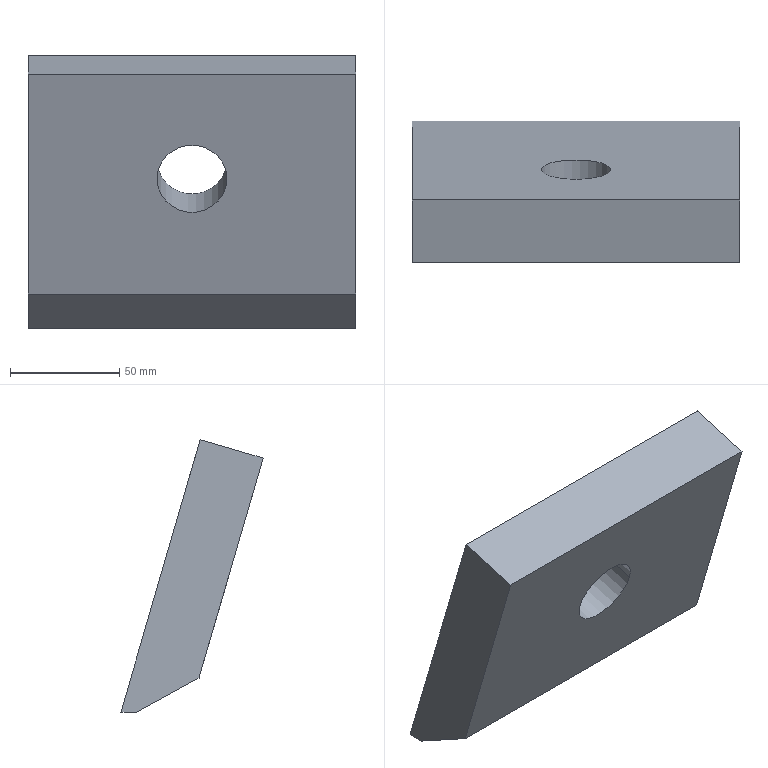Component | SolidWorks | Oslona ploca izbacivaca-4 | 1 solid | 9 faces | box 150 x 65.17 x 124.91 mm | volume 513260 mm3 | plane 6 | cylinder 3 | commonest cylinder face diameters 32 x2 521 x1
build123d program:
from build123d import *

# Parameters (mm, degrees)
SKETCH1_W           = 150
SKETCH1_H           = 130
SKETCH1_R           = 16
BOSS_EXTRUDE1_DEPTH = 30
CHAMFER1_SIZE       = 25
PIPECOPE_DEPTH      = 201.749
PIPECOPE_DEPTH_BACK = 201.749
PIPECOPESKETCH_R    = 260.5


with BuildPart() as part:
    # Sketch1 → Boss-Extrude1 (new body)
    with BuildSketch(Plane.XY):
        with Locations((75, 65)):
            Rectangle(SKETCH1_W, SKETCH1_H)
        with Locations((75, 80)):
            Circle(SKETCH1_R, mode=Mode.SUBTRACT)
    extrude(amount=BOSS_EXTRUDE1_DEPTH)

    # Chamfer1
    chamfer1_edges = [part.edges().sort_by_distance(p)[0] for p in [
        (75, 0, 0),
    ]]
    chamfer(chamfer1_edges, length=CHAMFER1_SIZE)

    # PipeCopeSketch → PipeCope (cut, two sides: drawn at the far end of the back side and taken through both)
    with BuildSketch(Plane(origin=(0, 0, 0), x_dir=(0, 0, -1), z_dir=(1, 0, 0)).offset(-PIPECOPE_DEPTH_BACK)):
        with Locations((42.874, -250.099)):
            Circle(PIPECOPESKETCH_R)
    extrude(amount=PIPECOPE_DEPTH + PIPECOPE_DEPTH_BACK, mode=Mode.SUBTRACT)


solid = part.part

# Placed as in the assembly
solid = solid.moved(Location((0.0002347, -28.803, 252.108), (-73.755, 0, 180)))
STEP:
#1=COLOUR_RGB('',0.7922,0.8196,0.9333);
#2=FILL_AREA_STYLE_COLOUR('',#1);
#3=FILL_AREA_STYLE('',(#2));
#4=SURFACE_STYLE_FILL_AREA(#3);
#5=SURFACE_SIDE_STYLE('',(#4));
#6=SURFACE_STYLE_USAGE(.BOTH.,#5);
#7=PRESENTATION_STYLE_ASSIGNMENT((#6));
#8=CARTESIAN_POINT('',(-2.323,-0.8811,13.28));
#9=VERTEX_POINT('',#8);
#10=CARTESIAN_POINT('',(-3.583,-0.8811,13.28));
#11=VERTEX_POINT('',#10);
#12=CARTESIAN_POINT('',(-2.953,-0.8811,13.28));
#13=DIRECTION('',(0.,0.9601,0.2797));
#14=DIRECTION('',(-1.,0.,0.));
#15=AXIS2_PLACEMENT_3D('',#12,#13,#14);
#16=CIRCLE('',#15,0.6299);
#17=EDGE_CURVE('',#9,#11,#16,.T.);
#18=ORIENTED_EDGE('',*,*,#17,.T.);
#19=CARTESIAN_POINT('',(-3.583,-2.015,12.949));
#20=VERTEX_POINT('',#19);
#21=CARTESIAN_POINT('',(-3.583,-0.8811,13.28));
#22=DIRECTION('',(-0.,-0.9601,-0.2797));
#23=VECTOR('',#22,39.37);
#24=LINE('',#21,#23);
#25=EDGE_CURVE('',#11,#20,#24,.T.);
#26=ORIENTED_EDGE('',*,*,#25,.T.);
#27=CARTESIAN_POINT('',(-2.323,-2.015,12.949));
#28=VERTEX_POINT('',#27);
#29=CARTESIAN_POINT('',(-2.953,-2.015,12.949));
#30=DIRECTION('',(0.,0.9601,0.2797));
#31=DIRECTION('',(-1.,0.,0.));
#32=AXIS2_PLACEMENT_3D('',#29,#30,#31);
#33=CIRCLE('',#32,0.6299);
#34=EDGE_CURVE('',#28,#20,#33,.T.);
#35=ORIENTED_EDGE('',*,*,#34,.F.);
#36=CARTESIAN_POINT('',(-2.323,-0.8811,13.28));
#37=DIRECTION('',(-0.,-0.9601,-0.2797));
#38=VECTOR('',#37,39.37);
#39=LINE('',#36,#38);
#40=EDGE_CURVE('',#9,#28,#39,.T.);
#41=ORIENTED_EDGE('',*,*,#40,.F.);
#42=EDGE_LOOP('',(#18,#26,#35,#41));
#43=FACE_OUTER_BOUND('',#42,.T.);
#44=CARTESIAN_POINT('',(-2.953,-0.8811,13.28));
#45=DIRECTION('',(-0.,-0.9601,-0.2797));
#46=DIRECTION('',(1.,0.,0.));
#47=AXIS2_PLACEMENT_3D('',#44,#45,#46);
#48=CYLINDRICAL_SURFACE('',#47,0.6299);
#49=ADVANCED_FACE('',(#43),#48,.F.);
#50=CARTESIAN_POINT('',(-5.906,-0.2823,10.252));
#51=VERTEX_POINT('',#50);
#52=CARTESIAN_POINT('',(-5.906,-0.00000001,10.256));
#53=VERTEX_POINT('',#52);
#54=CARTESIAN_POINT('',(-5.906,-0.,-0.));
#55=DIRECTION('',(-1.,0.,-0.));
#56=DIRECTION('',(0.,-0.9601,-0.2797));
#57=AXIS2_PLACEMENT_3D('',#54,#55,#56);
#58=CIRCLE('',#57,10.256);
#59=EDGE_CURVE('',#51,#53,#58,.T.);
#60=ORIENTED_EDGE('',*,*,#59,.F.);
#61=CARTESIAN_POINT('',(-5.906,-1.409,10.87));
#62=VERTEX_POINT('',#61);
#63=CARTESIAN_POINT('',(-5.906,-0.189,10.201));
#64=DIRECTION('',(-0.,-0.8767,0.4811));
#65=VECTOR('',#64,39.37);
#66=LINE('',#63,#65);
#67=EDGE_CURVE('',#51,#62,#66,.T.);
#68=ORIENTED_EDGE('',*,*,#67,.T.);
#69=CARTESIAN_POINT('',(-5.906,-2.566,14.839));
#70=VERTEX_POINT('',#69);
#71=CARTESIAN_POINT('',(-5.906,-1.134,9.925));
#72=DIRECTION('',(-0.,-0.2797,0.9601));
#73=VECTOR('',#72,39.37);
#74=LINE('',#71,#73);
#75=EDGE_CURVE('',#62,#70,#74,.T.);
#76=ORIENTED_EDGE('',*,*,#75,.T.);
#77=CARTESIAN_POINT('',(-5.906,-1.432,15.17));
#78=VERTEX_POINT('',#77);
#79=CARTESIAN_POINT('',(-5.906,-1.432,15.17));
#80=DIRECTION('',(-0.,-0.9601,-0.2797));
#81=VECTOR('',#80,39.37);
#82=LINE('',#79,#81);
#83=EDGE_CURVE('',#78,#70,#82,.T.);
#84=ORIENTED_EDGE('',*,*,#83,.F.);
#85=CARTESIAN_POINT('',(-5.906,-0.,10.256));
#86=DIRECTION('',(-0.,-0.2797,0.9601));
#87=VECTOR('',#86,39.37);
#88=LINE('',#85,#87);
#89=EDGE_CURVE('',#53,#78,#88,.T.);
#90=ORIENTED_EDGE('',*,*,#89,.F.);
#91=EDGE_LOOP('',(#60,#68,#76,#84,#90));
#92=FACE_OUTER_BOUND('',#91,.T.);
#93=CARTESIAN_POINT('',(-5.906,-0.,10.256));
#94=DIRECTION('',(1.,-0.,0.));
#95=DIRECTION('',(0.,0.9601,0.2797));
#96=AXIS2_PLACEMENT_3D('',#93,#94,#95);
#97=PLANE('',#96);
#98=ADVANCED_FACE('',(#92),#97,.F.);
#99=CARTESIAN_POINT('',(-0.,-1.432,15.17));
#100=VERTEX_POINT('',#99);
#101=CARTESIAN_POINT('',(0.00000047,-0.00001699,10.256));
#102=VERTEX_POINT('',#101);
#103=CARTESIAN_POINT('',(0.,-0.,10.256));
#104=DIRECTION('',(0.,0.2797,-0.9601));
#105=VECTOR('',#104,39.37);
#106=LINE('',#103,#105);
#107=EDGE_CURVE('',#100,#102,#106,.T.);
#108=ORIENTED_EDGE('',*,*,#107,.T.);
#109=CARTESIAN_POINT('',(0.,-0.,10.256));
#110=DIRECTION('',(-1.,0.,-0.));
#111=VECTOR('',#110,39.37);
#112=LINE('',#109,#111);
#113=EDGE_CURVE('',#102,#53,#112,.T.);
#114=ORIENTED_EDGE('',*,*,#113,.T.);
#115=ORIENTED_EDGE('',*,*,#89,.T.);
#116=CARTESIAN_POINT('',(-0.,-1.432,15.17));
#117=DIRECTION('',(1.,-0.,0.));
#118=VECTOR('',#117,39.37);
#119=LINE('',#116,#118);
#120=EDGE_CURVE('',#78,#100,#119,.T.);
#121=ORIENTED_EDGE('',*,*,#120,.T.);
#122=EDGE_LOOP('',(#108,#114,#115,#121));
#123=FACE_OUTER_BOUND('',#122,.T.);
#124=ORIENTED_EDGE('',*,*,#17,.F.);
#125=CARTESIAN_POINT('',(-2.953,-0.8811,13.28));
#126=DIRECTION('',(0.,0.9601,0.2797));
#127=DIRECTION('',(-1.,0.,0.));
#128=AXIS2_PLACEMENT_3D('',#125,#126,#127);
#129=CIRCLE('',#128,0.6299);
#130=EDGE_CURVE('',#11,#9,#129,.T.);
#131=ORIENTED_EDGE('',*,*,#130,.F.);
#132=EDGE_LOOP('',(#124,#131));
#133=FACE_BOUND('',#132,.T.);
#134=CARTESIAN_POINT('',(0.,-0.,10.256));
#135=DIRECTION('',(-0.,-0.9601,-0.2797));
#136=DIRECTION('',(1.,-0.,0.));
#137=AXIS2_PLACEMENT_3D('',#134,#135,#136);
#138=PLANE('',#137);
#139=ADVANCED_FACE('',(#123,#133),#138,.F.);
#140=ORIENTED_EDGE('',*,*,#75,.F.);
#141=CARTESIAN_POINT('',(-0.,-1.409,10.87));
#142=VERTEX_POINT('',#141);
#143=CARTESIAN_POINT('',(-0.,-1.409,10.87));
#144=DIRECTION('',(1.,-0.,0.));
#145=VECTOR('',#144,39.37);
#146=LINE('',#143,#145);
#147=EDGE_CURVE('',#62,#142,#146,.T.);
#148=ORIENTED_EDGE('',*,*,#147,.T.);
#149=CARTESIAN_POINT('',(-0.,-2.566,14.839));
#150=VERTEX_POINT('',#149);
#151=CARTESIAN_POINT('',(-0.,-1.134,9.925));
#152=DIRECTION('',(0.,0.2797,-0.9601));
#153=VECTOR('',#152,39.37);
#154=LINE('',#151,#153);
#155=EDGE_CURVE('',#150,#142,#154,.T.);
#156=ORIENTED_EDGE('',*,*,#155,.F.);
#157=CARTESIAN_POINT('',(-0.,-2.566,14.839));
#158=DIRECTION('',(1.,-0.,0.));
#159=VECTOR('',#158,39.37);
#160=LINE('',#157,#159);
#161=EDGE_CURVE('',#70,#150,#160,.T.);
#162=ORIENTED_EDGE('',*,*,#161,.F.);
#163=EDGE_LOOP('',(#140,#148,#156,#162));
#164=FACE_OUTER_BOUND('',#163,.T.);
#165=ORIENTED_EDGE('',*,*,#34,.T.);
#166=CARTESIAN_POINT('',(-2.953,-2.015,12.949));
#167=DIRECTION('',(0.,0.9601,0.2797));
#168=DIRECTION('',(-1.,0.,0.));
#169=AXIS2_PLACEMENT_3D('',#166,#167,#168);
#170=CIRCLE('',#169,0.6299);
#171=EDGE_CURVE('',#20,#28,#170,.T.);
#172=ORIENTED_EDGE('',*,*,#171,.T.);
#173=EDGE_LOOP('',(#165,#172));
#174=FACE_BOUND('',#173,.T.);
#175=CARTESIAN_POINT('',(-0.,-1.134,9.925));
#176=DIRECTION('',(-0.,-0.9601,-0.2797));
#177=DIRECTION('',(1.,-0.,0.));
#178=AXIS2_PLACEMENT_3D('',#175,#176,#177);
#179=PLANE('',#178);
#180=ADVANCED_FACE('',(#164,#174),#179,.T.);
#181=CARTESIAN_POINT('',(0.00000047,-0.2823,10.252));
#182=VERTEX_POINT('',#181);
#183=CARTESIAN_POINT('',(-0.,-0.189,10.201));
#184=DIRECTION('',(0.,0.8767,-0.4811));
#185=VECTOR('',#184,39.37);
#186=LINE('',#183,#185);
#187=EDGE_CURVE('',#142,#182,#186,.T.);
#188=ORIENTED_EDGE('',*,*,#187,.T.);
#189=CARTESIAN_POINT('',(0.00000047,-0.2823,10.252));
#190=CARTESIAN_POINT('',(-0.,-0.2353,10.253));
#191=CARTESIAN_POINT('',(-0.,-0.1412,10.255));
#192=CARTESIAN_POINT('',(-0.,-0.04709,10.256));
#193=CARTESIAN_POINT('',(0.00000047,-0.00001699,10.256));
#194=B_SPLINE_CURVE_WITH_KNOTS('',3,(#189,#190,#191,#192,#193),.UNSPECIFIED.,.F.,.F.,(4,1,4),(0.2907,0.2929,0.2951),.UNSPECIFIED.);
#195=EDGE_CURVE('',#182,#102,#194,.T.);
#196=ORIENTED_EDGE('',*,*,#195,.T.);
#197=ORIENTED_EDGE('',*,*,#107,.F.);
#198=CARTESIAN_POINT('',(-0.,-1.432,15.17));
#199=DIRECTION('',(-0.,-0.9601,-0.2797));
#200=VECTOR('',#199,39.37);
#201=LINE('',#198,#200);
#202=EDGE_CURVE('',#100,#150,#201,.T.);
#203=ORIENTED_EDGE('',*,*,#202,.T.);
#204=ORIENTED_EDGE('',*,*,#155,.T.);
#205=EDGE_LOOP('',(#188,#196,#197,#203,#204));
#206=FACE_OUTER_BOUND('',#205,.T.);
#207=CARTESIAN_POINT('',(0.,-0.,10.256));
#208=DIRECTION('',(-1.,0.,-0.));
#209=DIRECTION('',(-0.,-0.9601,-0.2797));
#210=AXIS2_PLACEMENT_3D('',#207,#208,#209);
#211=PLANE('',#210);
#212=ADVANCED_FACE('',(#206),#211,.F.);
#213=ORIENTED_EDGE('',*,*,#161,.T.);
#214=ORIENTED_EDGE('',*,*,#202,.F.);
#215=ORIENTED_EDGE('',*,*,#120,.F.);
#216=ORIENTED_EDGE('',*,*,#83,.T.);
#217=EDGE_LOOP('',(#213,#214,#215,#216));
#218=FACE_OUTER_BOUND('',#217,.T.);
#219=CARTESIAN_POINT('',(-0.,-1.432,15.17));
#220=DIRECTION('',(0.,0.2797,-0.9601));
#221=DIRECTION('',(-0.,-0.9601,-0.2797));
#222=AXIS2_PLACEMENT_3D('',#219,#220,#221);
#223=PLANE('',#222);
#224=ADVANCED_FACE('',(#218),#223,.F.);
#225=ORIENTED_EDGE('',*,*,#25,.F.);
#226=ORIENTED_EDGE('',*,*,#130,.T.);
#227=ORIENTED_EDGE('',*,*,#40,.T.);
#228=ORIENTED_EDGE('',*,*,#171,.F.);
#229=EDGE_LOOP('',(#225,#226,#227,#228));
#230=FACE_OUTER_BOUND('',#229,.T.);
#231=CARTESIAN_POINT('',(-2.953,-0.8811,13.28));
#232=DIRECTION('',(-0.,-0.9601,-0.2797));
#233=DIRECTION('',(1.,0.,0.));
#234=AXIS2_PLACEMENT_3D('',#231,#232,#233);
#235=CYLINDRICAL_SURFACE('',#234,0.6299);
#236=ADVANCED_FACE('',(#230),#235,.F.);
#237=CARTESIAN_POINT('',(0.00000047,-0.2823,10.252));
#238=DIRECTION('',(-1.,0.,-0.));
#239=VECTOR('',#238,39.37);
#240=LINE('',#237,#239);
#241=EDGE_CURVE('',#182,#51,#240,.T.);
#242=ORIENTED_EDGE('',*,*,#241,.F.);
#243=ORIENTED_EDGE('',*,*,#187,.F.);
#244=ORIENTED_EDGE('',*,*,#147,.F.);
#245=ORIENTED_EDGE('',*,*,#67,.F.);
#246=EDGE_LOOP('',(#242,#243,#244,#245));
#247=FACE_OUTER_BOUND('',#246,.T.);
#248=CARTESIAN_POINT('',(-0.,-0.189,10.201));
#249=DIRECTION('',(0.,-0.4811,-0.8767));
#250=DIRECTION('',(1.,-0.,0.));
#251=AXIS2_PLACEMENT_3D('',#248,#249,#250);
#252=PLANE('',#251);
#253=ADVANCED_FACE('',(#247),#252,.T.);
#254=ORIENTED_EDGE('',*,*,#195,.F.);
#255=ORIENTED_EDGE('',*,*,#241,.T.);
#256=ORIENTED_EDGE('',*,*,#59,.T.);
#257=ORIENTED_EDGE('',*,*,#113,.F.);
#258=EDGE_LOOP('',(#254,#255,#256,#257));
#259=FACE_OUTER_BOUND('',#258,.T.);
#260=CARTESIAN_POINT('',(0.00000047,-0.,-0.));
#261=DIRECTION('',(-1.,0.,-0.));
#262=DIRECTION('',(-0.,-0.9601,-0.2797));
#263=AXIS2_PLACEMENT_3D('',#260,#261,#262);
#264=CYLINDRICAL_SURFACE('',#263,10.256);
#265=ADVANCED_FACE('',(#259),#264,.F.);
#266=CLOSED_SHELL('',(#49,#98,#139,#180,#212,#224,#236,#253,#265));
#267=MANIFOLD_SOLID_BREP('',#266);
#268=STYLED_ITEM('',(#7),#267);
#269=(LENGTH_UNIT()NAMED_UNIT(*)SI_UNIT($,.METRE.));
#270=LENGTH_MEASURE_WITH_UNIT(LENGTH_MEASURE(0.0254),#269);
#271=DIMENSIONAL_EXPONENTS(1.,0.,0.,0.,0.,0.,0.);
#272=(CONVERSION_BASED_UNIT('',#270)LENGTH_UNIT()NAMED_UNIT(#271));
#273=UNCERTAINTY_MEASURE_WITH_UNIT(LENGTH_MEASURE(0.00001),#272,'','');
#274=(NAMED_UNIT(*)PLANE_ANGLE_UNIT()SI_UNIT($,.RADIAN.));
#275=(NAMED_UNIT(*)SI_UNIT($,.STERADIAN.)SOLID_ANGLE_UNIT());
#276=(GEOMETRIC_REPRESENTATION_CONTEXT(3)GLOBAL_UNCERTAINTY_ASSIGNED_CONTEXT((#273))GLOBAL_UNIT_ASSIGNED_CONTEXT((#272,#274,#275))REPRESENTATION_CONTEXT('',''));
#277=MECHANICAL_DESIGN_GEOMETRIC_PRESENTATION_REPRESENTATION('',(#268),#276);
#278=PRESENTATION_LAYER_ASSIGNMENT('','',(#268));
#279=CARTESIAN_POINT('',(0.,0.,0.));
#280=DIRECTION('',(0.,0.,1.));
#281=DIRECTION('',(1.,0.,0.));
#282=AXIS2_PLACEMENT_3D('',#279,#280,#281);
#283=(LENGTH_UNIT()NAMED_UNIT(*)SI_UNIT($,.METRE.));
#284=LENGTH_MEASURE_WITH_UNIT(LENGTH_MEASURE(0.0254),#283);
#285=DIMENSIONAL_EXPONENTS(1.,0.,0.,0.,0.,0.,0.);
#286=(CONVERSION_BASED_UNIT('',#284)LENGTH_UNIT()NAMED_UNIT(#285));
#287=UNCERTAINTY_MEASURE_WITH_UNIT(LENGTH_MEASURE(0.00001),#286,'','');
#288=(NAMED_UNIT(*)PLANE_ANGLE_UNIT()SI_UNIT($,.RADIAN.));
#289=(NAMED_UNIT(*)SI_UNIT($,.STERADIAN.)SOLID_ANGLE_UNIT());
#290=(GEOMETRIC_REPRESENTATION_CONTEXT(3)GLOBAL_UNCERTAINTY_ASSIGNED_CONTEXT((#287))GLOBAL_UNIT_ASSIGNED_CONTEXT((#286,#288,#289))REPRESENTATION_CONTEXT('',''));
#291=ADVANCED_BREP_SHAPE_REPRESENTATION('',(#267,#282),#290);